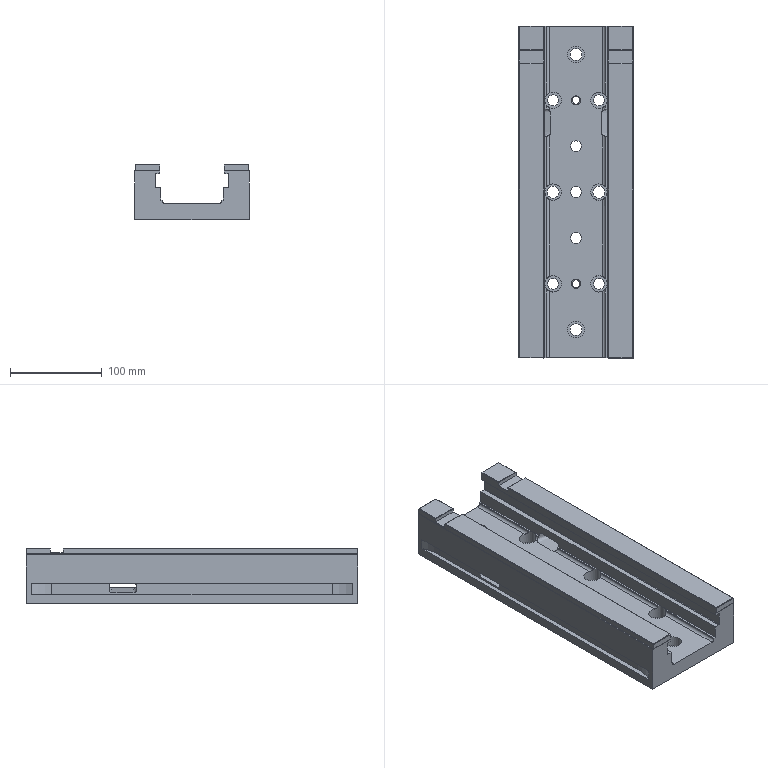Component | NX | CLAMP_BODY_1 | 1 solid | 138 faces | volume 1487779 mm3 | plane 86 | cylinder 48 | cone 2 | spline 2 | commonest cylinder face diameters 6 x10 1 x10 12 x8 18 x8 13 x4 100 x4 8.5 x2 25 x2